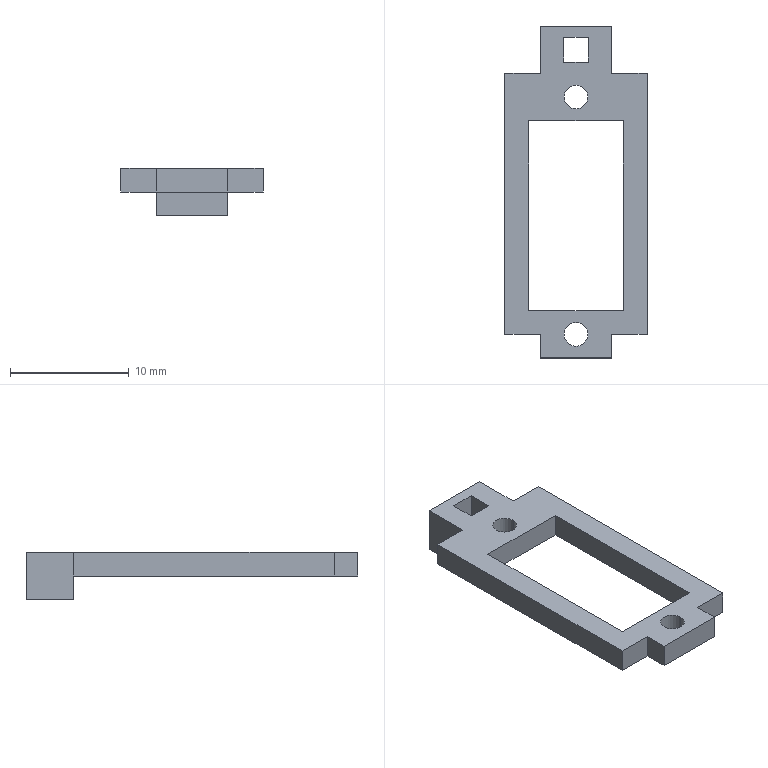Component | SolidWorks | ServoHanger-1 | 1 solid | 28 faces | box 12 x 28 x 4 mm | volume 362 mm3 | plane 24 | cylinder 4 | commonest cylinder face diameters 2 x4
build123d program:
from build123d import *

# Parameters (mm, degrees)
SKETCH1_W           = 6
SKETCH1_H           = 4
SKETCH1_W_2         = 2.1
SKETCH1_H_2         = 2.1
BOSS_EXTRUDE1_DEPTH = 4
SKETCH2_W           = 6
SKETCH2_H           = 24
BOSS_EXTRUDE2_DEPTH = 2
SKETCH3_R           = 1
CUT_EXTRUDE1_DEPTH  = 2
SKETCH5_W           = 3
SKETCH5_H           = 24
BOSS_EXTRUDE3_DEPTH = 2
SKETCH4_W           = 8
SKETCH4_H           = 16
CUT_EXTRUDE2_DEPTH  = 2
SKETCH6_W           = 3
SKETCH6_H           = 2
CUT_EXTRUDE3_DEPTH  = 2


with BuildPart() as part:
    # Sketch1 → Boss-Extrude1 (new body)
    with BuildSketch(Plane.XY):
        Rectangle(SKETCH1_W, SKETCH1_H)
        Rectangle(SKETCH1_W_2, SKETCH1_H_2, mode=Mode.SUBTRACT)
    extrude(amount=BOSS_EXTRUDE1_DEPTH)

    # Sketch2 → Boss-Extrude2 (add)
    with BuildSketch(Plane.XY.offset(4)):
        with Locations((0, -14)):
            Rectangle(SKETCH2_W, SKETCH2_H)
    extrude(amount=-BOSS_EXTRUDE2_DEPTH)

    # Sketch3 → Cut-Extrude1 (cut)
    with BuildSketch(Plane.XY.offset(4)):
        with Locations((0, -4)):
            Circle(SKETCH3_R)
        with Locations(Location((0, -24, 0), (0, 0, 180))):
            Circle(SKETCH3_R)
    extrude(amount=-CUT_EXTRUDE1_DEPTH, mode=Mode.SUBTRACT)

    # Sketch5 → Boss-Extrude3 (add)
    with BuildSketch(Plane(origin=(0, 0, 2), x_dir=(-1, 0, 0), z_dir=(0, 0, -1))):
        with Locations((-4.5, -14)):
            Rectangle(SKETCH5_W, SKETCH5_H)
        with Locations((4.5, -14)):
            Rectangle(SKETCH5_W, SKETCH5_H)
    extrude(amount=-BOSS_EXTRUDE3_DEPTH)

    # Sketch4 → Cut-Extrude2 (cut)
    with BuildSketch(Plane(origin=(0, 0, 2), x_dir=(-1, 0, 0), z_dir=(0, 0, -1))):
        with Locations((0, -14)):
            Rectangle(SKETCH4_W, SKETCH4_H)
    extrude(amount=-CUT_EXTRUDE2_DEPTH, mode=Mode.SUBTRACT)

    # Sketch6 → Cut-Extrude3 (cut)
    with BuildSketch(Plane.XY.offset(4)):
        with Locations((-4.5, -25)):
            Rectangle(SKETCH6_W, SKETCH6_H)
    cut_extrude3 = extrude(amount=-CUT_EXTRUDE3_DEPTH, mode=Mode.SUBTRACT)

    # Mirror1: Cut-Extrude3 across plane
    add(cut_extrude3.mirror(Plane(origin=(0, 0, 0), x_dir=(0, 0, 1), z_dir=(1, 0, 0))), mode=Mode.SUBTRACT)


solid = part.part

# Placed as in the assembly
solid = solid.moved(Location((0.5986, 8.796, -71.03), (0, 0, 0)))
STEP:
#1=COLOUR_RGB('',0.7922,0.8196,0.9333);
#2=FILL_AREA_STYLE_COLOUR('',#1);
#3=FILL_AREA_STYLE('',(#2));
#4=SURFACE_STYLE_FILL_AREA(#3);
#5=SURFACE_SIDE_STYLE('',(#4));
#6=SURFACE_STYLE_USAGE(.BOTH.,#5);
#7=PRESENTATION_STYLE_ASSIGNMENT((#6));
#8=CARTESIAN_POINT('',(-0.0158,0.1888,-2.718));
#9=VERTEX_POINT('',#8);
#10=CARTESIAN_POINT('',(0.06294,0.1888,-2.718));
#11=VERTEX_POINT('',#10);
#12=CARTESIAN_POINT('',(0.02357,0.1888,-2.718));
#13=DIRECTION('',(0.,0.,1.));
#14=DIRECTION('',(1.,0.,0.));
#15=AXIS2_PLACEMENT_3D('',#12,#13,#14);
#16=CIRCLE('',#15,0.03937);
#17=EDGE_CURVE('',#9,#11,#16,.T.);
#18=ORIENTED_EDGE('',*,*,#17,.F.);
#19=CARTESIAN_POINT('',(-0.0158,0.1888,-2.639));
#20=VERTEX_POINT('',#19);
#21=CARTESIAN_POINT('',(-0.0158,0.1888,-2.718));
#22=DIRECTION('',(0.,0.,1.));
#23=VECTOR('',#22,39.37);
#24=LINE('',#21,#23);
#25=EDGE_CURVE('',#9,#20,#24,.T.);
#26=ORIENTED_EDGE('',*,*,#25,.T.);
#27=CARTESIAN_POINT('',(0.06294,0.1888,-2.639));
#28=VERTEX_POINT('',#27);
#29=CARTESIAN_POINT('',(0.02357,0.1888,-2.639));
#30=DIRECTION('',(0.,0.,1.));
#31=DIRECTION('',(1.,0.,0.));
#32=AXIS2_PLACEMENT_3D('',#29,#30,#31);
#33=CIRCLE('',#32,0.03937);
#34=EDGE_CURVE('',#20,#28,#33,.T.);
#35=ORIENTED_EDGE('',*,*,#34,.T.);
#36=CARTESIAN_POINT('',(0.06294,0.1888,-2.718));
#37=DIRECTION('',(0.,0.,1.));
#38=VECTOR('',#37,39.37);
#39=LINE('',#36,#38);
#40=EDGE_CURVE('',#11,#28,#39,.T.);
#41=ORIENTED_EDGE('',*,*,#40,.F.);
#42=EDGE_LOOP('',(#18,#26,#35,#41));
#43=FACE_OUTER_BOUND('',#42,.T.);
#44=CARTESIAN_POINT('',(0.02357,0.1888,-2.718));
#45=DIRECTION('',(0.,0.,1.));
#46=DIRECTION('',(1.,0.,0.));
#47=AXIS2_PLACEMENT_3D('',#44,#45,#46);
#48=CYLINDRICAL_SURFACE('',#47,0.03937);
#49=ADVANCED_FACE('',(#43),#48,.F.);
#50=CARTESIAN_POINT('',(-0.0158,-0.5986,-2.718));
#51=VERTEX_POINT('',#50);
#52=CARTESIAN_POINT('',(0.06294,-0.5986,-2.718));
#53=VERTEX_POINT('',#52);
#54=CARTESIAN_POINT('',(0.02357,-0.5986,-2.718));
#55=DIRECTION('',(0.,0.,1.));
#56=DIRECTION('',(-1.,0.,0.));
#57=AXIS2_PLACEMENT_3D('',#54,#55,#56);
#58=CIRCLE('',#57,0.03937);
#59=EDGE_CURVE('',#51,#53,#58,.T.);
#60=ORIENTED_EDGE('',*,*,#59,.F.);
#61=CARTESIAN_POINT('',(-0.0158,-0.5986,-2.639));
#62=VERTEX_POINT('',#61);
#63=CARTESIAN_POINT('',(-0.0158,-0.5986,-2.718));
#64=DIRECTION('',(0.,0.,1.));
#65=VECTOR('',#64,39.37);
#66=LINE('',#63,#65);
#67=EDGE_CURVE('',#51,#62,#66,.T.);
#68=ORIENTED_EDGE('',*,*,#67,.T.);
#69=CARTESIAN_POINT('',(0.06294,-0.5986,-2.639));
#70=VERTEX_POINT('',#69);
#71=CARTESIAN_POINT('',(0.02357,-0.5986,-2.639));
#72=DIRECTION('',(0.,0.,1.));
#73=DIRECTION('',(-1.,0.,0.));
#74=AXIS2_PLACEMENT_3D('',#71,#72,#73);
#75=CIRCLE('',#74,0.03937);
#76=EDGE_CURVE('',#62,#70,#75,.T.);
#77=ORIENTED_EDGE('',*,*,#76,.T.);
#78=CARTESIAN_POINT('',(0.06294,-0.5986,-2.718));
#79=DIRECTION('',(0.,0.,1.));
#80=VECTOR('',#79,39.37);
#81=LINE('',#78,#80);
#82=EDGE_CURVE('',#53,#70,#81,.T.);
#83=ORIENTED_EDGE('',*,*,#82,.F.);
#84=EDGE_LOOP('',(#60,#68,#77,#83));
#85=FACE_OUTER_BOUND('',#84,.T.);
#86=CARTESIAN_POINT('',(0.02357,-0.5986,-2.718));
#87=DIRECTION('',(0.,0.,1.));
#88=DIRECTION('',(1.,0.,0.));
#89=AXIS2_PLACEMENT_3D('',#86,#87,#88);
#90=CYLINDRICAL_SURFACE('',#89,0.03937);
#91=ADVANCED_FACE('',(#85),#90,.F.);
#92=CARTESIAN_POINT('',(0.06491,0.305,-2.639));
#93=VERTEX_POINT('',#92);
#94=CARTESIAN_POINT('',(0.06491,0.3876,-2.639));
#95=VERTEX_POINT('',#94);
#96=CARTESIAN_POINT('',(0.06491,0.305,-2.639));
#97=DIRECTION('',(0.,1.,0.));
#98=VECTOR('',#97,39.37);
#99=LINE('',#96,#98);
#100=EDGE_CURVE('',#93,#95,#99,.T.);
#101=ORIENTED_EDGE('',*,*,#100,.F.);
#102=CARTESIAN_POINT('',(-0.01777,0.305,-2.639));
#103=VERTEX_POINT('',#102);
#104=CARTESIAN_POINT('',(-0.01777,0.305,-2.639));
#105=DIRECTION('',(1.,0.,0.));
#106=VECTOR('',#105,39.37);
#107=LINE('',#104,#106);
#108=EDGE_CURVE('',#103,#93,#107,.T.);
#109=ORIENTED_EDGE('',*,*,#108,.F.);
#110=CARTESIAN_POINT('',(-0.01777,0.3876,-2.639));
#111=VERTEX_POINT('',#110);
#112=CARTESIAN_POINT('',(-0.01777,0.305,-2.639));
#113=DIRECTION('',(0.,-1.,0.));
#114=VECTOR('',#113,39.37);
#115=LINE('',#112,#114);
#116=EDGE_CURVE('',#111,#103,#115,.T.);
#117=ORIENTED_EDGE('',*,*,#116,.F.);
#118=CARTESIAN_POINT('',(-0.01777,0.3876,-2.639));
#119=DIRECTION('',(-1.,0.,0.));
#120=VECTOR('',#119,39.37);
#121=LINE('',#118,#120);
#122=EDGE_CURVE('',#95,#111,#121,.T.);
#123=ORIENTED_EDGE('',*,*,#122,.F.);
#124=EDGE_LOOP('',(#101,#109,#117,#123));
#125=FACE_BOUND('',#124,.T.);
#126=CARTESIAN_POINT('',(0.02357,-0.5986,-2.639));
#127=DIRECTION('',(0.,0.,1.));
#128=DIRECTION('',(-1.,0.,0.));
#129=AXIS2_PLACEMENT_3D('',#126,#127,#128);
#130=CIRCLE('',#129,0.03937);
#131=EDGE_CURVE('',#70,#62,#130,.T.);
#132=ORIENTED_EDGE('',*,*,#131,.F.);
#133=ORIENTED_EDGE('',*,*,#76,.F.);
#134=EDGE_LOOP('',(#132,#133));
#135=FACE_BOUND('',#134,.T.);
#136=CARTESIAN_POINT('',(0.02357,0.1888,-2.639));
#137=DIRECTION('',(0.,0.,1.));
#138=DIRECTION('',(1.,0.,0.));
#139=AXIS2_PLACEMENT_3D('',#136,#137,#138);
#140=CIRCLE('',#139,0.03937);
#141=EDGE_CURVE('',#28,#20,#140,.T.);
#142=ORIENTED_EDGE('',*,*,#141,.F.);
#143=ORIENTED_EDGE('',*,*,#34,.F.);
#144=EDGE_LOOP('',(#142,#143));
#145=FACE_BOUND('',#144,.T.);
#146=CARTESIAN_POINT('',(-0.1339,0.1101,-2.639));
#147=VERTEX_POINT('',#146);
#148=CARTESIAN_POINT('',(0.181,0.1101,-2.639));
#149=VERTEX_POINT('',#148);
#150=CARTESIAN_POINT('',(0.181,0.1101,-2.639));
#151=DIRECTION('',(1.,0.,0.));
#152=VECTOR('',#151,39.37);
#153=LINE('',#150,#152);
#154=EDGE_CURVE('',#147,#149,#153,.T.);
#155=ORIENTED_EDGE('',*,*,#154,.T.);
#156=CARTESIAN_POINT('',(0.181,-0.5198,-2.639));
#157=VERTEX_POINT('',#156);
#158=CARTESIAN_POINT('',(0.181,-0.5198,-2.639));
#159=DIRECTION('',(0.,-1.,0.));
#160=VECTOR('',#159,39.37);
#161=LINE('',#158,#160);
#162=EDGE_CURVE('',#149,#157,#161,.T.);
#163=ORIENTED_EDGE('',*,*,#162,.T.);
#164=CARTESIAN_POINT('',(-0.1339,-0.5198,-2.639));
#165=VERTEX_POINT('',#164);
#166=CARTESIAN_POINT('',(0.181,-0.5198,-2.639));
#167=DIRECTION('',(-1.,0.,0.));
#168=VECTOR('',#167,39.37);
#169=LINE('',#166,#168);
#170=EDGE_CURVE('',#157,#165,#169,.T.);
#171=ORIENTED_EDGE('',*,*,#170,.T.);
#172=CARTESIAN_POINT('',(-0.1339,-0.5198,-2.639));
#173=DIRECTION('',(0.,1.,0.));
#174=VECTOR('',#173,39.37);
#175=LINE('',#172,#174);
#176=EDGE_CURVE('',#165,#147,#175,.T.);
#177=ORIENTED_EDGE('',*,*,#176,.T.);
#178=EDGE_LOOP('',(#155,#163,#171,#177));
#179=FACE_BOUND('',#178,.T.);
#180=CARTESIAN_POINT('',(0.1417,-0.6773,-2.639));
#181=VERTEX_POINT('',#180);
#182=CARTESIAN_POINT('',(0.1417,-0.5986,-2.639));
#183=VERTEX_POINT('',#182);
#184=CARTESIAN_POINT('',(0.1417,-0.6773,-2.639));
#185=DIRECTION('',(0.,1.,0.));
#186=VECTOR('',#185,39.37);
#187=LINE('',#184,#186);
#188=EDGE_CURVE('',#181,#183,#187,.T.);
#189=ORIENTED_EDGE('',*,*,#188,.T.);
#190=CARTESIAN_POINT('',(0.2598,-0.5986,-2.639));
#191=VERTEX_POINT('',#190);
#192=CARTESIAN_POINT('',(0.2598,-0.5986,-2.639));
#193=DIRECTION('',(1.,0.,0.));
#194=VECTOR('',#193,39.37);
#195=LINE('',#192,#194);
#196=EDGE_CURVE('',#183,#191,#195,.T.);
#197=ORIENTED_EDGE('',*,*,#196,.T.);
#198=CARTESIAN_POINT('',(0.2598,0.2676,-2.639));
#199=VERTEX_POINT('',#198);
#200=CARTESIAN_POINT('',(0.2598,0.2676,-2.639));
#201=DIRECTION('',(0.,1.,0.));
#202=VECTOR('',#201,39.37);
#203=LINE('',#200,#202);
#204=EDGE_CURVE('',#191,#199,#203,.T.);
#205=ORIENTED_EDGE('',*,*,#204,.T.);
#206=CARTESIAN_POINT('',(0.1417,0.2676,-2.639));
#207=VERTEX_POINT('',#206);
#208=CARTESIAN_POINT('',(0.1417,0.2676,-2.639));
#209=DIRECTION('',(-1.,0.,0.));
#210=VECTOR('',#209,39.37);
#211=LINE('',#208,#210);
#212=EDGE_CURVE('',#199,#207,#211,.T.);
#213=ORIENTED_EDGE('',*,*,#212,.T.);
#214=CARTESIAN_POINT('',(0.1417,0.425,-2.639));
#215=VERTEX_POINT('',#214);
#216=CARTESIAN_POINT('',(0.1417,0.2676,-2.639));
#217=DIRECTION('',(0.,1.,0.));
#218=VECTOR('',#217,39.37);
#219=LINE('',#216,#218);
#220=EDGE_CURVE('',#207,#215,#219,.T.);
#221=ORIENTED_EDGE('',*,*,#220,.T.);
#222=CARTESIAN_POINT('',(-0.09454,0.425,-2.639));
#223=VERTEX_POINT('',#222);
#224=CARTESIAN_POINT('',(-0.09454,0.425,-2.639));
#225=DIRECTION('',(-1.,0.,0.));
#226=VECTOR('',#225,39.37);
#227=LINE('',#224,#226);
#228=EDGE_CURVE('',#215,#223,#227,.T.);
#229=ORIENTED_EDGE('',*,*,#228,.T.);
#230=CARTESIAN_POINT('',(-0.09454,0.2676,-2.639));
#231=VERTEX_POINT('',#230);
#232=CARTESIAN_POINT('',(-0.09454,0.2676,-2.639));
#233=DIRECTION('',(0.,-1.,0.));
#234=VECTOR('',#233,39.37);
#235=LINE('',#232,#234);
#236=EDGE_CURVE('',#223,#231,#235,.T.);
#237=ORIENTED_EDGE('',*,*,#236,.T.);
#238=CARTESIAN_POINT('',(-0.2127,0.2676,-2.639));
#239=VERTEX_POINT('',#238);
#240=CARTESIAN_POINT('',(-0.09454,0.2676,-2.639));
#241=DIRECTION('',(-1.,0.,0.));
#242=VECTOR('',#241,39.37);
#243=LINE('',#240,#242);
#244=EDGE_CURVE('',#231,#239,#243,.T.);
#245=ORIENTED_EDGE('',*,*,#244,.T.);
#246=CARTESIAN_POINT('',(-0.2127,-0.5986,-2.639));
#247=VERTEX_POINT('',#246);
#248=CARTESIAN_POINT('',(-0.2127,0.2676,-2.639));
#249=DIRECTION('',(-0.,-1.,0.));
#250=VECTOR('',#249,39.37);
#251=LINE('',#248,#250);
#252=EDGE_CURVE('',#239,#247,#251,.T.);
#253=ORIENTED_EDGE('',*,*,#252,.T.);
#254=CARTESIAN_POINT('',(-0.09454,-0.5986,-2.639));
#255=VERTEX_POINT('',#254);
#256=CARTESIAN_POINT('',(-0.2127,-0.5986,-2.639));
#257=DIRECTION('',(-1.,0.,0.));
#258=VECTOR('',#257,39.37);
#259=LINE('',#256,#258);
#260=EDGE_CURVE('',#255,#247,#259,.T.);
#261=ORIENTED_EDGE('',*,*,#260,.F.);
#262=CARTESIAN_POINT('',(-0.09454,-0.6773,-2.639));
#263=VERTEX_POINT('',#262);
#264=CARTESIAN_POINT('',(-0.09454,-0.6773,-2.639));
#265=DIRECTION('',(0.,1.,0.));
#266=VECTOR('',#265,39.37);
#267=LINE('',#264,#266);
#268=EDGE_CURVE('',#263,#255,#267,.T.);
#269=ORIENTED_EDGE('',*,*,#268,.F.);
#270=CARTESIAN_POINT('',(-0.09454,-0.6773,-2.639));
#271=DIRECTION('',(1.,0.,0.));
#272=VECTOR('',#271,39.37);
#273=LINE('',#270,#272);
#274=EDGE_CURVE('',#263,#181,#273,.T.);
#275=ORIENTED_EDGE('',*,*,#274,.T.);
#276=EDGE_LOOP('',(#189,#197,#205,#213,#221,#229,#237,#245,#253,#261,#269,#275));
#277=FACE_OUTER_BOUND('',#276,.T.);
#278=CARTESIAN_POINT('',(0.02357,0.3463,-2.639));
#279=DIRECTION('',(0.,0.,-1.));
#280=DIRECTION('',(-1.,0.,0.));
#281=AXIS2_PLACEMENT_3D('',#278,#279,#280);
#282=PLANE('',#281);
#283=ADVANCED_FACE('',(#125,#135,#145,#179,#277),#282,.F.);
#284=CARTESIAN_POINT('',(-0.09454,-0.6773,-2.718));
#285=VERTEX_POINT('',#284);
#286=CARTESIAN_POINT('',(0.1417,-0.6773,-2.718));
#287=VERTEX_POINT('',#286);
#288=CARTESIAN_POINT('',(-0.09454,-0.6773,-2.718));
#289=DIRECTION('',(1.,0.,0.));
#290=VECTOR('',#289,39.37);
#291=LINE('',#288,#290);
#292=EDGE_CURVE('',#285,#287,#291,.T.);
#293=ORIENTED_EDGE('',*,*,#292,.T.);
#294=CARTESIAN_POINT('',(0.1417,-0.6773,-2.718));
#295=DIRECTION('',(0.,0.,1.));
#296=VECTOR('',#295,39.37);
#297=LINE('',#294,#296);
#298=EDGE_CURVE('',#287,#181,#297,.T.);
#299=ORIENTED_EDGE('',*,*,#298,.T.);
#300=ORIENTED_EDGE('',*,*,#274,.F.);
#301=CARTESIAN_POINT('',(-0.09454,-0.6773,-2.718));
#302=DIRECTION('',(0.,0.,1.));
#303=VECTOR('',#302,39.37);
#304=LINE('',#301,#303);
#305=EDGE_CURVE('',#285,#263,#304,.T.);
#306=ORIENTED_EDGE('',*,*,#305,.F.);
#307=EDGE_LOOP('',(#293,#299,#300,#306));
#308=FACE_OUTER_BOUND('',#307,.T.);
#309=CARTESIAN_POINT('',(-0.09454,-0.6773,-2.718));
#310=DIRECTION('',(0.,-1.,0.));
#311=DIRECTION('',(0.,0.,-1.));
#312=AXIS2_PLACEMENT_3D('',#309,#310,#311);
#313=PLANE('',#312);
#314=ADVANCED_FACE('',(#308),#313,.T.);
#315=CARTESIAN_POINT('',(0.02357,-0.5986,-2.718));
#316=DIRECTION('',(0.,0.,1.));
#317=DIRECTION('',(-1.,0.,0.));
#318=AXIS2_PLACEMENT_3D('',#315,#316,#317);
#319=CIRCLE('',#318,0.03937);
#320=EDGE_CURVE('',#53,#51,#319,.T.);
#321=ORIENTED_EDGE('',*,*,#320,.T.);
#322=ORIENTED_EDGE('',*,*,#59,.T.);
#323=EDGE_LOOP('',(#321,#322));
#324=FACE_BOUND('',#323,.T.);
#325=CARTESIAN_POINT('',(0.02357,0.1888,-2.718));
#326=DIRECTION('',(0.,0.,1.));
#327=DIRECTION('',(1.,0.,0.));
#328=AXIS2_PLACEMENT_3D('',#325,#326,#327);
#329=CIRCLE('',#328,0.03937);
#330=EDGE_CURVE('',#11,#9,#329,.T.);
#331=ORIENTED_EDGE('',*,*,#330,.T.);
#332=ORIENTED_EDGE('',*,*,#17,.T.);
#333=EDGE_LOOP('',(#331,#332));
#334=FACE_BOUND('',#333,.T.);
#335=CARTESIAN_POINT('',(0.181,-0.5198,-2.718));
#336=VERTEX_POINT('',#335);
#337=CARTESIAN_POINT('',(-0.1339,-0.5198,-2.718));
#338=VERTEX_POINT('',#337);
#339=CARTESIAN_POINT('',(0.181,-0.5198,-2.718));
#340=DIRECTION('',(-1.,0.,0.));
#341=VECTOR('',#340,39.37);
#342=LINE('',#339,#341);
#343=EDGE_CURVE('',#336,#338,#342,.T.);
#344=ORIENTED_EDGE('',*,*,#343,.F.);
#345=CARTESIAN_POINT('',(0.181,0.1101,-2.718));
#346=VERTEX_POINT('',#345);
#347=CARTESIAN_POINT('',(0.181,-0.5198,-2.718));
#348=DIRECTION('',(0.,-1.,0.));
#349=VECTOR('',#348,39.37);
#350=LINE('',#347,#349);
#351=EDGE_CURVE('',#346,#336,#350,.T.);
#352=ORIENTED_EDGE('',*,*,#351,.F.);
#353=CARTESIAN_POINT('',(-0.1339,0.1101,-2.718));
#354=VERTEX_POINT('',#353);
#355=CARTESIAN_POINT('',(0.181,0.1101,-2.718));
#356=DIRECTION('',(1.,0.,0.));
#357=VECTOR('',#356,39.37);
#358=LINE('',#355,#357);
#359=EDGE_CURVE('',#354,#346,#358,.T.);
#360=ORIENTED_EDGE('',*,*,#359,.F.);
#361=CARTESIAN_POINT('',(-0.1339,-0.5198,-2.718));
#362=DIRECTION('',(0.,1.,0.));
#363=VECTOR('',#362,39.37);
#364=LINE('',#361,#363);
#365=EDGE_CURVE('',#338,#354,#364,.T.);
#366=ORIENTED_EDGE('',*,*,#365,.F.);
#367=EDGE_LOOP('',(#344,#352,#360,#366));
#368=FACE_BOUND('',#367,.T.);
#369=CARTESIAN_POINT('',(0.1417,-0.5986,-2.718));
#370=VERTEX_POINT('',#369);
#371=CARTESIAN_POINT('',(0.1417,-0.6773,-2.718));
#372=DIRECTION('',(0.,1.,0.));
#373=VECTOR('',#372,39.37);
#374=LINE('',#371,#373);
#375=EDGE_CURVE('',#287,#370,#374,.T.);
#376=ORIENTED_EDGE('',*,*,#375,.F.);
#377=ORIENTED_EDGE('',*,*,#292,.F.);
#378=CARTESIAN_POINT('',(-0.09454,-0.5986,-2.718));
#379=VERTEX_POINT('',#378);
#380=CARTESIAN_POINT('',(-0.09454,-0.6773,-2.718));
#381=DIRECTION('',(0.,1.,0.));
#382=VECTOR('',#381,39.37);
#383=LINE('',#380,#382);
#384=EDGE_CURVE('',#285,#379,#383,.T.);
#385=ORIENTED_EDGE('',*,*,#384,.T.);
#386=CARTESIAN_POINT('',(-0.2127,-0.5986,-2.718));
#387=VERTEX_POINT('',#386);
#388=CARTESIAN_POINT('',(-0.2127,-0.5986,-2.718));
#389=DIRECTION('',(-1.,0.,0.));
#390=VECTOR('',#389,39.37);
#391=LINE('',#388,#390);
#392=EDGE_CURVE('',#379,#387,#391,.T.);
#393=ORIENTED_EDGE('',*,*,#392,.T.);
#394=CARTESIAN_POINT('',(-0.2127,0.2676,-2.718));
#395=VERTEX_POINT('',#394);
#396=CARTESIAN_POINT('',(-0.2127,0.2676,-2.718));
#397=DIRECTION('',(0.,1.,0.));
#398=VECTOR('',#397,39.37);
#399=LINE('',#396,#398);
#400=EDGE_CURVE('',#387,#395,#399,.T.);
#401=ORIENTED_EDGE('',*,*,#400,.T.);
#402=CARTESIAN_POINT('',(-0.09454,0.2676,-2.718));
#403=VERTEX_POINT('',#402);
#404=CARTESIAN_POINT('',(-0.09454,0.2676,-2.718));
#405=DIRECTION('',(1.,-0.,0.));
#406=VECTOR('',#405,39.37);
#407=LINE('',#404,#406);
#408=EDGE_CURVE('',#395,#403,#407,.T.);
#409=ORIENTED_EDGE('',*,*,#408,.T.);
#410=CARTESIAN_POINT('',(0.1417,0.2676,-2.718));
#411=VERTEX_POINT('',#410);
#412=CARTESIAN_POINT('',(-0.09454,0.2676,-2.718));
#413=DIRECTION('',(-1.,0.,0.));
#414=VECTOR('',#413,39.37);
#415=LINE('',#412,#414);
#416=EDGE_CURVE('',#411,#403,#415,.T.);
#417=ORIENTED_EDGE('',*,*,#416,.F.);
#418=CARTESIAN_POINT('',(0.2598,0.2676,-2.718));
#419=VERTEX_POINT('',#418);
#420=CARTESIAN_POINT('',(0.1417,0.2676,-2.718));
#421=DIRECTION('',(1.,0.,0.));
#422=VECTOR('',#421,39.37);
#423=LINE('',#420,#422);
#424=EDGE_CURVE('',#411,#419,#423,.T.);
#425=ORIENTED_EDGE('',*,*,#424,.T.);
#426=CARTESIAN_POINT('',(0.2598,-0.5986,-2.718));
#427=VERTEX_POINT('',#426);
#428=CARTESIAN_POINT('',(0.2598,0.2676,-2.718));
#429=DIRECTION('',(-0.,-1.,0.));
#430=VECTOR('',#429,39.37);
#431=LINE('',#428,#430);
#432=EDGE_CURVE('',#419,#427,#431,.T.);
#433=ORIENTED_EDGE('',*,*,#432,.T.);
#434=CARTESIAN_POINT('',(0.2598,-0.5986,-2.718));
#435=DIRECTION('',(1.,0.,0.));
#436=VECTOR('',#435,39.37);
#437=LINE('',#434,#436);
#438=EDGE_CURVE('',#370,#427,#437,.T.);
#439=ORIENTED_EDGE('',*,*,#438,.F.);
#440=EDGE_LOOP('',(#376,#377,#385,#393,#401,#409,#417,#425,#433,#439));
#441=FACE_OUTER_BOUND('',#440,.T.);
#442=CARTESIAN_POINT('',(0.02357,0.3463,-2.718));
#443=DIRECTION('',(0.,0.,1.));
#444=DIRECTION('',(1.,0.,0.));
#445=AXIS2_PLACEMENT_3D('',#442,#443,#444);
#446=PLANE('',#445);
#447=ADVANCED_FACE('',(#324,#334,#368,#441),#446,.F.);
#448=ORIENTED_EDGE('',*,*,#204,.F.);
#449=CARTESIAN_POINT('',(0.2598,-0.5986,-2.718));
#450=DIRECTION('',(0.,0.,1.));
#451=VECTOR('',#450,39.37);
#452=LINE('',#449,#451);
#453=EDGE_CURVE('',#427,#191,#452,.T.);
#454=ORIENTED_EDGE('',*,*,#453,.F.);
#455=ORIENTED_EDGE('',*,*,#432,.F.);
#456=CARTESIAN_POINT('',(0.2598,0.2676,-1.687));
#457=DIRECTION('',(0.,0.,-1.));
#458=VECTOR('',#457,39.37);
#459=LINE('',#456,#458);
#460=EDGE_CURVE('',#199,#419,#459,.T.);
#461=ORIENTED_EDGE('',*,*,#460,.F.);
#462=EDGE_LOOP('',(#448,#454,#455,#461));
#463=FACE_OUTER_BOUND('',#462,.T.);
#464=CARTESIAN_POINT('',(0.2598,0.2676,-1.687));
#465=DIRECTION('',(1.,-0.,0.));
#466=DIRECTION('',(0.,1.,0.));
#467=AXIS2_PLACEMENT_3D('',#464,#465,#466);
#468=PLANE('',#467);
#469=ADVANCED_FACE('',(#463),#468,.T.);
#470=CARTESIAN_POINT('',(-0.09454,0.2676,-1.687));
#471=DIRECTION('',(0.,0.,-1.));
#472=VECTOR('',#471,39.37);
#473=LINE('',#470,#472);
#474=EDGE_CURVE('',#231,#403,#473,.T.);
#475=ORIENTED_EDGE('',*,*,#474,.F.);
#476=ORIENTED_EDGE('',*,*,#236,.F.);
#477=CARTESIAN_POINT('',(-0.09454,0.425,-2.796));
#478=VERTEX_POINT('',#477);
#479=CARTESIAN_POINT('',(-0.09454,0.425,-2.639));
#480=DIRECTION('',(0.,0.,-1.));
#481=VECTOR('',#480,39.37);
#482=LINE('',#479,#481);
#483=EDGE_CURVE('',#223,#478,#482,.T.);
#484=ORIENTED_EDGE('',*,*,#483,.T.);
#485=CARTESIAN_POINT('',(-0.09454,0.2676,-2.796));
#486=VERTEX_POINT('',#485);
#487=CARTESIAN_POINT('',(-0.09454,0.2676,-2.796));
#488=DIRECTION('',(0.,-1.,0.));
#489=VECTOR('',#488,39.37);
#490=LINE('',#487,#489);
#491=EDGE_CURVE('',#478,#486,#490,.T.);
#492=ORIENTED_EDGE('',*,*,#491,.T.);
#493=CARTESIAN_POINT('',(-0.09454,0.2676,-2.639));
#494=DIRECTION('',(0.,0.,-1.));
#495=VECTOR('',#494,39.37);
#496=LINE('',#493,#495);
#497=EDGE_CURVE('',#403,#486,#496,.T.);
#498=ORIENTED_EDGE('',*,*,#497,.F.);
#499=EDGE_LOOP('',(#475,#476,#484,#492,#498));
#500=FACE_OUTER_BOUND('',#499,.T.);
#501=CARTESIAN_POINT('',(-0.09454,0.2676,-2.639));
#502=DIRECTION('',(1.,0.,0.));
#503=DIRECTION('',(0.,0.,-1.));
#504=AXIS2_PLACEMENT_3D('',#501,#502,#503);
#505=PLANE('',#504);
#506=ADVANCED_FACE('',(#500),#505,.F.);
#507=CARTESIAN_POINT('',(0.1417,0.2676,-2.796));
#508=VERTEX_POINT('',#507);
#509=CARTESIAN_POINT('',(0.1417,0.425,-2.796));
#510=VERTEX_POINT('',#509);
#511=CARTESIAN_POINT('',(0.1417,0.2676,-2.796));
#512=DIRECTION('',(0.,1.,0.));
#513=VECTOR('',#512,39.37);
#514=LINE('',#511,#513);
#515=EDGE_CURVE('',#508,#510,#514,.T.);
#516=ORIENTED_EDGE('',*,*,#515,.F.);
#517=CARTESIAN_POINT('',(-0.09454,0.2676,-2.796));
#518=DIRECTION('',(1.,0.,0.));
#519=VECTOR('',#518,39.37);
#520=LINE('',#517,#519);
#521=EDGE_CURVE('',#486,#508,#520,.T.);
#522=ORIENTED_EDGE('',*,*,#521,.F.);
#523=ORIENTED_EDGE('',*,*,#491,.F.);
#524=CARTESIAN_POINT('',(-0.09454,0.425,-2.796));
#525=DIRECTION('',(-1.,0.,0.));
#526=VECTOR('',#525,39.37);
#527=LINE('',#524,#526);
#528=EDGE_CURVE('',#510,#478,#527,.T.);
#529=ORIENTED_EDGE('',*,*,#528,.F.);
#530=EDGE_LOOP('',(#516,#522,#523,#529));
#531=FACE_OUTER_BOUND('',#530,.T.);
#532=CARTESIAN_POINT('',(-0.01777,0.305,-2.796));
#533=VERTEX_POINT('',#532);
#534=CARTESIAN_POINT('',(0.06491,0.305,-2.796));
#535=VERTEX_POINT('',#534);
#536=CARTESIAN_POINT('',(-0.01777,0.305,-2.796));
#537=DIRECTION('',(1.,0.,0.));
#538=VECTOR('',#537,39.37);
#539=LINE('',#536,#538);
#540=EDGE_CURVE('',#533,#535,#539,.T.);
#541=ORIENTED_EDGE('',*,*,#540,.T.);
#542=CARTESIAN_POINT('',(0.06491,0.3876,-2.796));
#543=VERTEX_POINT('',#542);
#544=CARTESIAN_POINT('',(0.06491,0.305,-2.796));
#545=DIRECTION('',(0.,1.,0.));
#546=VECTOR('',#545,39.37);
#547=LINE('',#544,#546);
#548=EDGE_CURVE('',#535,#543,#547,.T.);
#549=ORIENTED_EDGE('',*,*,#548,.T.);
#550=CARTESIAN_POINT('',(-0.01777,0.3876,-2.796));
#551=VERTEX_POINT('',#550);
#552=CARTESIAN_POINT('',(-0.01777,0.3876,-2.796));
#553=DIRECTION('',(-1.,0.,0.));
#554=VECTOR('',#553,39.37);
#555=LINE('',#552,#554);
#556=EDGE_CURVE('',#543,#551,#555,.T.);
#557=ORIENTED_EDGE('',*,*,#556,.T.);
#558=CARTESIAN_POINT('',(-0.01777,0.305,-2.796));
#559=DIRECTION('',(0.,-1.,0.));
#560=VECTOR('',#559,39.37);
#561=LINE('',#558,#560);
#562=EDGE_CURVE('',#551,#533,#561,.T.);
#563=ORIENTED_EDGE('',*,*,#562,.T.);
#564=EDGE_LOOP('',(#541,#549,#557,#563));
#565=FACE_BOUND('',#564,.T.);
#566=CARTESIAN_POINT('',(0.02357,0.3463,-2.796));
#567=DIRECTION('',(0.,0.,-1.));
#568=DIRECTION('',(-1.,0.,0.));
#569=AXIS2_PLACEMENT_3D('',#566,#567,#568);
#570=PLANE('',#569);
#571=ADVANCED_FACE('',(#531,#565),#570,.T.);
#572=ORIENTED_EDGE('',*,*,#220,.F.);
#573=CARTESIAN_POINT('',(0.1417,0.2676,-1.687));
#574=DIRECTION('',(0.,0.,-1.));
#575=VECTOR('',#574,39.37);
#576=LINE('',#573,#575);
#577=EDGE_CURVE('',#207,#411,#576,.T.);
#578=ORIENTED_EDGE('',*,*,#577,.T.);
#579=CARTESIAN_POINT('',(0.1417,0.2676,-2.639));
#580=DIRECTION('',(0.,0.,-1.));
#581=VECTOR('',#580,39.37);
#582=LINE('',#579,#581);
#583=EDGE_CURVE('',#411,#508,#582,.T.);
#584=ORIENTED_EDGE('',*,*,#583,.T.);
#585=ORIENTED_EDGE('',*,*,#515,.T.);
#586=CARTESIAN_POINT('',(0.1417,0.425,-2.639));
#587=DIRECTION('',(0.,0.,-1.));
#588=VECTOR('',#587,39.37);
#589=LINE('',#586,#588);
#590=EDGE_CURVE('',#215,#510,#589,.T.);
#591=ORIENTED_EDGE('',*,*,#590,.F.);
#592=EDGE_LOOP('',(#572,#578,#584,#585,#591));
#593=FACE_OUTER_BOUND('',#592,.T.);
#594=CARTESIAN_POINT('',(0.1417,0.2676,-2.639));
#595=DIRECTION('',(-1.,0.,0.));
#596=DIRECTION('',(0.,0.,1.));
#597=AXIS2_PLACEMENT_3D('',#594,#595,#596);
#598=PLANE('',#597);
#599=ADVANCED_FACE('',(#593),#598,.F.);
#600=ORIENTED_EDGE('',*,*,#528,.T.);
#601=ORIENTED_EDGE('',*,*,#483,.F.);
#602=ORIENTED_EDGE('',*,*,#228,.F.);
#603=ORIENTED_EDGE('',*,*,#590,.T.);
#604=EDGE_LOOP('',(#600,#601,#602,#603));
#605=FACE_OUTER_BOUND('',#604,.T.);
#606=CARTESIAN_POINT('',(-0.09454,0.425,-2.639));
#607=DIRECTION('',(0.,-1.,0.));
#608=DIRECTION('',(0.,0.,-1.));
#609=AXIS2_PLACEMENT_3D('',#606,#607,#608);
#610=PLANE('',#609);
#611=ADVANCED_FACE('',(#605),#610,.F.);
#612=ORIENTED_EDGE('',*,*,#583,.F.);
#613=ORIENTED_EDGE('',*,*,#416,.T.);
#614=ORIENTED_EDGE('',*,*,#497,.T.);
#615=ORIENTED_EDGE('',*,*,#521,.T.);
#616=EDGE_LOOP('',(#612,#613,#614,#615));
#617=FACE_OUTER_BOUND('',#616,.T.);
#618=CARTESIAN_POINT('',(-0.09454,0.2676,-2.639));
#619=DIRECTION('',(0.,1.,0.));
#620=DIRECTION('',(0.,0.,1.));
#621=AXIS2_PLACEMENT_3D('',#618,#619,#620);
#622=PLANE('',#621);
#623=ADVANCED_FACE('',(#617),#622,.F.);
#624=ORIENTED_EDGE('',*,*,#548,.F.);
#625=CARTESIAN_POINT('',(0.06491,0.305,-2.639));
#626=DIRECTION('',(0.,0.,-1.));
#627=VECTOR('',#626,39.37);
#628=LINE('',#625,#627);
#629=EDGE_CURVE('',#93,#535,#628,.T.);
#630=ORIENTED_EDGE('',*,*,#629,.F.);
#631=ORIENTED_EDGE('',*,*,#100,.T.);
#632=CARTESIAN_POINT('',(0.06491,0.3876,-2.639));
#633=DIRECTION('',(0.,0.,-1.));
#634=VECTOR('',#633,39.37);
#635=LINE('',#632,#634);
#636=EDGE_CURVE('',#95,#543,#635,.T.);
#637=ORIENTED_EDGE('',*,*,#636,.T.);
#638=EDGE_LOOP('',(#624,#630,#631,#637));
#639=FACE_OUTER_BOUND('',#638,.T.);
#640=CARTESIAN_POINT('',(0.06491,0.305,-2.639));
#641=DIRECTION('',(-1.,0.,0.));
#642=DIRECTION('',(0.,0.,1.));
#643=AXIS2_PLACEMENT_3D('',#640,#641,#642);
#644=PLANE('',#643);
#645=ADVANCED_FACE('',(#639),#644,.T.);
#646=ORIENTED_EDGE('',*,*,#556,.F.);
#647=ORIENTED_EDGE('',*,*,#636,.F.);
#648=ORIENTED_EDGE('',*,*,#122,.T.);
#649=CARTESIAN_POINT('',(-0.01777,0.3876,-2.639));
#650=DIRECTION('',(0.,0.,-1.));
#651=VECTOR('',#650,39.37);
#652=LINE('',#649,#651);
#653=EDGE_CURVE('',#111,#551,#652,.T.);
#654=ORIENTED_EDGE('',*,*,#653,.T.);
#655=EDGE_LOOP('',(#646,#647,#648,#654));
#656=FACE_OUTER_BOUND('',#655,.T.);
#657=CARTESIAN_POINT('',(-0.01777,0.3876,-2.639));
#658=DIRECTION('',(0.,-1.,0.));
#659=DIRECTION('',(0.,0.,-1.));
#660=AXIS2_PLACEMENT_3D('',#657,#658,#659);
#661=PLANE('',#660);
#662=ADVANCED_FACE('',(#656),#661,.T.);
#663=ORIENTED_EDGE('',*,*,#562,.F.);
#664=ORIENTED_EDGE('',*,*,#653,.F.);
#665=ORIENTED_EDGE('',*,*,#116,.T.);
#666=CARTESIAN_POINT('',(-0.01777,0.305,-2.639));
#667=DIRECTION('',(0.,0.,-1.));
#668=VECTOR('',#667,39.37);
#669=LINE('',#666,#668);
#670=EDGE_CURVE('',#103,#533,#669,.T.);
#671=ORIENTED_EDGE('',*,*,#670,.T.);
#672=EDGE_LOOP('',(#663,#664,#665,#671));
#673=FACE_OUTER_BOUND('',#672,.T.);
#674=CARTESIAN_POINT('',(-0.01777,0.305,-2.639));
#675=DIRECTION('',(1.,0.,0.));
#676=DIRECTION('',(0.,0.,-1.));
#677=AXIS2_PLACEMENT_3D('',#674,#675,#676);
#678=PLANE('',#677);
#679=ADVANCED_FACE('',(#673),#678,.T.);
#680=ORIENTED_EDGE('',*,*,#540,.F.);
#681=ORIENTED_EDGE('',*,*,#670,.F.);
#682=ORIENTED_EDGE('',*,*,#108,.T.);
#683=ORIENTED_EDGE('',*,*,#629,.T.);
#684=EDGE_LOOP('',(#680,#681,#682,#683));
#685=FACE_OUTER_BOUND('',#684,.T.);
#686=CARTESIAN_POINT('',(-0.01777,0.305,-2.639));
#687=DIRECTION('',(0.,1.,0.));
#688=DIRECTION('',(0.,0.,1.));
#689=AXIS2_PLACEMENT_3D('',#686,#687,#688);
#690=PLANE('',#689);
#691=ADVANCED_FACE('',(#685),#690,.T.);
#692=ORIENTED_EDGE('',*,*,#67,.F.);
#693=ORIENTED_EDGE('',*,*,#320,.F.);
#694=ORIENTED_EDGE('',*,*,#82,.T.);
#695=ORIENTED_EDGE('',*,*,#131,.T.);
#696=EDGE_LOOP('',(#692,#693,#694,#695));
#697=FACE_OUTER_BOUND('',#696,.T.);
#698=CARTESIAN_POINT('',(0.02357,-0.5986,-2.718));
#699=DIRECTION('',(0.,0.,1.));
#700=DIRECTION('',(1.,0.,0.));
#701=AXIS2_PLACEMENT_3D('',#698,#699,#700);
#702=CYLINDRICAL_SURFACE('',#701,0.03937);
#703=ADVANCED_FACE('',(#697),#702,.F.);
#704=ORIENTED_EDGE('',*,*,#25,.F.);
#705=ORIENTED_EDGE('',*,*,#330,.F.);
#706=ORIENTED_EDGE('',*,*,#40,.T.);
#707=ORIENTED_EDGE('',*,*,#141,.T.);
#708=EDGE_LOOP('',(#704,#705,#706,#707));
#709=FACE_OUTER_BOUND('',#708,.T.);
#710=CARTESIAN_POINT('',(0.02357,0.1888,-2.718));
#711=DIRECTION('',(0.,0.,1.));
#712=DIRECTION('',(1.,0.,0.));
#713=AXIS2_PLACEMENT_3D('',#710,#711,#712);
#714=CYLINDRICAL_SURFACE('',#713,0.03937);
#715=ADVANCED_FACE('',(#709),#714,.F.);
#716=ORIENTED_EDGE('',*,*,#212,.F.);
#717=ORIENTED_EDGE('',*,*,#460,.T.);
#718=ORIENTED_EDGE('',*,*,#424,.F.);
#719=ORIENTED_EDGE('',*,*,#577,.F.);
#720=EDGE_LOOP('',(#716,#717,#718,#719));
#721=FACE_OUTER_BOUND('',#720,.T.);
#722=CARTESIAN_POINT('',(0.1417,0.2676,-1.687));
#723=DIRECTION('',(0.,1.,0.));
#724=DIRECTION('',(0.,0.,1.));
#725=AXIS2_PLACEMENT_3D('',#722,#723,#724);
#726=PLANE('',#725);
#727=ADVANCED_FACE('',(#721),#726,.T.);
#728=ORIENTED_EDGE('',*,*,#244,.F.);
#729=ORIENTED_EDGE('',*,*,#474,.T.);
#730=ORIENTED_EDGE('',*,*,#408,.F.);
#731=CARTESIAN_POINT('',(-0.2127,0.2676,-1.687));
#732=DIRECTION('',(0.,0.,-1.));
#733=VECTOR('',#732,39.37);
#734=LINE('',#731,#733);
#735=EDGE_CURVE('',#239,#395,#734,.T.);
#736=ORIENTED_EDGE('',*,*,#735,.F.);
#737=EDGE_LOOP('',(#728,#729,#730,#736));
#738=FACE_OUTER_BOUND('',#737,.T.);
#739=CARTESIAN_POINT('',(-0.09454,0.2676,-1.687));
#740=DIRECTION('',(0.,1.,0.));
#741=DIRECTION('',(-1.,0.,0.));
#742=AXIS2_PLACEMENT_3D('',#739,#740,#741);
#743=PLANE('',#742);
#744=ADVANCED_FACE('',(#738),#743,.T.);
#745=CARTESIAN_POINT('',(-0.2127,-0.5986,-2.718));
#746=DIRECTION('',(0.,0.,1.));
#747=VECTOR('',#746,39.37);
#748=LINE('',#745,#747);
#749=EDGE_CURVE('',#387,#247,#748,.T.);
#750=ORIENTED_EDGE('',*,*,#749,.T.);
#751=ORIENTED_EDGE('',*,*,#252,.F.);
#752=ORIENTED_EDGE('',*,*,#735,.T.);
#753=ORIENTED_EDGE('',*,*,#400,.F.);
#754=EDGE_LOOP('',(#750,#751,#752,#753));
#755=FACE_OUTER_BOUND('',#754,.T.);
#756=CARTESIAN_POINT('',(-0.2127,0.2676,-1.687));
#757=DIRECTION('',(-1.,0.,0.));
#758=DIRECTION('',(-0.,-1.,0.));
#759=AXIS2_PLACEMENT_3D('',#756,#757,#758);
#760=PLANE('',#759);
#761=ADVANCED_FACE('',(#755),#760,.T.);
#762=ORIENTED_EDGE('',*,*,#351,.T.);
#763=CARTESIAN_POINT('',(0.181,-0.5198,-2.639));
#764=DIRECTION('',(0.,0.,-1.));
#765=VECTOR('',#764,39.37);
#766=LINE('',#763,#765);
#767=EDGE_CURVE('',#157,#336,#766,.T.);
#768=ORIENTED_EDGE('',*,*,#767,.F.);
#769=ORIENTED_EDGE('',*,*,#162,.F.);
#770=CARTESIAN_POINT('',(0.181,0.1101,-2.639));
#771=DIRECTION('',(0.,0.,-1.));
#772=VECTOR('',#771,39.37);
#773=LINE('',#770,#772);
#774=EDGE_CURVE('',#149,#346,#773,.T.);
#775=ORIENTED_EDGE('',*,*,#774,.T.);
#776=EDGE_LOOP('',(#762,#768,#769,#775));
#777=FACE_OUTER_BOUND('',#776,.T.);
#778=CARTESIAN_POINT('',(0.181,-0.5198,-2.639));
#779=DIRECTION('',(1.,0.,0.));
#780=DIRECTION('',(0.,0.,-1.));
#781=AXIS2_PLACEMENT_3D('',#778,#779,#780);
#782=PLANE('',#781);
#783=ADVANCED_FACE('',(#777),#782,.F.);
#784=ORIENTED_EDGE('',*,*,#359,.T.);
#785=ORIENTED_EDGE('',*,*,#774,.F.);
#786=ORIENTED_EDGE('',*,*,#154,.F.);
#787=CARTESIAN_POINT('',(-0.1339,0.1101,-2.639));
#788=DIRECTION('',(0.,0.,-1.));
#789=VECTOR('',#788,39.37);
#790=LINE('',#787,#789);
#791=EDGE_CURVE('',#147,#354,#790,.T.);
#792=ORIENTED_EDGE('',*,*,#791,.T.);
#793=EDGE_LOOP('',(#784,#785,#786,#792));
#794=FACE_OUTER_BOUND('',#793,.T.);
#795=CARTESIAN_POINT('',(0.181,0.1101,-2.639));
#796=DIRECTION('',(0.,1.,0.));
#797=DIRECTION('',(0.,0.,1.));
#798=AXIS2_PLACEMENT_3D('',#795,#796,#797);
#799=PLANE('',#798);
#800=ADVANCED_FACE('',(#794),#799,.F.);
#801=ORIENTED_EDGE('',*,*,#365,.T.);
#802=ORIENTED_EDGE('',*,*,#791,.F.);
#803=ORIENTED_EDGE('',*,*,#176,.F.);
#804=CARTESIAN_POINT('',(-0.1339,-0.5198,-2.639));
#805=DIRECTION('',(0.,0.,-1.));
#806=VECTOR('',#805,39.37);
#807=LINE('',#804,#806);
#808=EDGE_CURVE('',#165,#338,#807,.T.);
#809=ORIENTED_EDGE('',*,*,#808,.T.);
#810=EDGE_LOOP('',(#801,#802,#803,#809));
#811=FACE_OUTER_BOUND('',#810,.T.);
#812=CARTESIAN_POINT('',(-0.1339,-0.5198,-2.639));
#813=DIRECTION('',(-1.,0.,0.));
#814=DIRECTION('',(0.,0.,1.));
#815=AXIS2_PLACEMENT_3D('',#812,#813,#814);
#816=PLANE('',#815);
#817=ADVANCED_FACE('',(#811),#816,.F.);
#818=ORIENTED_EDGE('',*,*,#343,.T.);
#819=ORIENTED_EDGE('',*,*,#808,.F.);
#820=ORIENTED_EDGE('',*,*,#170,.F.);
#821=ORIENTED_EDGE('',*,*,#767,.T.);
#822=EDGE_LOOP('',(#818,#819,#820,#821));
#823=FACE_OUTER_BOUND('',#822,.T.);
#824=CARTESIAN_POINT('',(0.181,-0.5198,-2.639));
#825=DIRECTION('',(0.,-1.,0.));
#826=DIRECTION('',(0.,0.,-1.));
#827=AXIS2_PLACEMENT_3D('',#824,#825,#826);
#828=PLANE('',#827);
#829=ADVANCED_FACE('',(#823),#828,.F.);
#830=ORIENTED_EDGE('',*,*,#260,.T.);
#831=ORIENTED_EDGE('',*,*,#749,.F.);
#832=ORIENTED_EDGE('',*,*,#392,.F.);
#833=CARTESIAN_POINT('',(-0.09454,-0.5986,-2.718));
#834=DIRECTION('',(0.,0.,1.));
#835=VECTOR('',#834,39.37);
#836=LINE('',#833,#835);
#837=EDGE_CURVE('',#379,#255,#836,.T.);
#838=ORIENTED_EDGE('',*,*,#837,.T.);
#839=EDGE_LOOP('',(#830,#831,#832,#838));
#840=FACE_OUTER_BOUND('',#839,.T.);
#841=CARTESIAN_POINT('',(-0.2127,-0.5986,-2.718));
#842=DIRECTION('',(0.,1.,0.));
#843=DIRECTION('',(0.,0.,1.));
#844=AXIS2_PLACEMENT_3D('',#841,#842,#843);
#845=PLANE('',#844);
#846=ADVANCED_FACE('',(#840),#845,.F.);
#847=ORIENTED_EDGE('',*,*,#268,.T.);
#848=ORIENTED_EDGE('',*,*,#837,.F.);
#849=ORIENTED_EDGE('',*,*,#384,.F.);
#850=ORIENTED_EDGE('',*,*,#305,.T.);
#851=EDGE_LOOP('',(#847,#848,#849,#850));
#852=FACE_OUTER_BOUND('',#851,.T.);
#853=CARTESIAN_POINT('',(-0.09454,-0.6773,-2.718));
#854=DIRECTION('',(1.,0.,0.));
#855=DIRECTION('',(0.,0.,-1.));
#856=AXIS2_PLACEMENT_3D('',#853,#854,#855);
#857=PLANE('',#856);
#858=ADVANCED_FACE('',(#852),#857,.F.);
#859=ORIENTED_EDGE('',*,*,#188,.F.);
#860=ORIENTED_EDGE('',*,*,#298,.F.);
#861=ORIENTED_EDGE('',*,*,#375,.T.);
#862=CARTESIAN_POINT('',(0.1417,-0.5986,-2.718));
#863=DIRECTION('',(0.,0.,1.));
#864=VECTOR('',#863,39.37);
#865=LINE('',#862,#864);
#866=EDGE_CURVE('',#370,#183,#865,.T.);
#867=ORIENTED_EDGE('',*,*,#866,.T.);
#868=EDGE_LOOP('',(#859,#860,#861,#867));
#869=FACE_OUTER_BOUND('',#868,.T.);
#870=CARTESIAN_POINT('',(0.1417,-0.6773,-2.718));
#871=DIRECTION('',(1.,0.,0.));
#872=DIRECTION('',(0.,0.,-1.));
#873=AXIS2_PLACEMENT_3D('',#870,#871,#872);
#874=PLANE('',#873);
#875=ADVANCED_FACE('',(#869),#874,.T.);
#876=ORIENTED_EDGE('',*,*,#196,.F.);
#877=ORIENTED_EDGE('',*,*,#866,.F.);
#878=ORIENTED_EDGE('',*,*,#438,.T.);
#879=ORIENTED_EDGE('',*,*,#453,.T.);
#880=EDGE_LOOP('',(#876,#877,#878,#879));
#881=FACE_OUTER_BOUND('',#880,.T.);
#882=CARTESIAN_POINT('',(0.2598,-0.5986,-2.718));
#883=DIRECTION('',(0.,-1.,0.));
#884=DIRECTION('',(0.,0.,-1.));
#885=AXIS2_PLACEMENT_3D('',#882,#883,#884);
#886=PLANE('',#885);
#887=ADVANCED_FACE('',(#881),#886,.T.);
#888=CLOSED_SHELL('',(#49,#91,#283,#314,#447,#469,#506,#571,#599,#611,#623,#645,#662,#679,#691,#703,#715,#727,#744,#761,#783,#800,#817,#829,#846,#858,#875,#887));
#889=MANIFOLD_SOLID_BREP('',#888);
#890=STYLED_ITEM('',(#7),#889);
#891=(LENGTH_UNIT()NAMED_UNIT(*)SI_UNIT($,.METRE.));
#892=LENGTH_MEASURE_WITH_UNIT(LENGTH_MEASURE(0.0254),#891);
#893=DIMENSIONAL_EXPONENTS(1.,0.,0.,0.,0.,0.,0.);
#894=(CONVERSION_BASED_UNIT('',#892)LENGTH_UNIT()NAMED_UNIT(#893));
#895=UNCERTAINTY_MEASURE_WITH_UNIT(LENGTH_MEASURE(0.00001),#894,'','');
#896=(NAMED_UNIT(*)PLANE_ANGLE_UNIT()SI_UNIT($,.RADIAN.));
#897=(NAMED_UNIT(*)SI_UNIT($,.STERADIAN.)SOLID_ANGLE_UNIT());
#898=(GEOMETRIC_REPRESENTATION_CONTEXT(3)GLOBAL_UNCERTAINTY_ASSIGNED_CONTEXT((#895))GLOBAL_UNIT_ASSIGNED_CONTEXT((#894,#896,#897))REPRESENTATION_CONTEXT('',''));
#899=MECHANICAL_DESIGN_GEOMETRIC_PRESENTATION_REPRESENTATION('',(#890),#898);
#900=CARTESIAN_POINT('',(0.,0.,0.));
#901=DIRECTION('',(0.,0.,1.));
#902=DIRECTION('',(1.,0.,0.));
#903=AXIS2_PLACEMENT_3D('',#900,#901,#902);
#904=(LENGTH_UNIT()NAMED_UNIT(*)SI_UNIT($,.METRE.));
#905=LENGTH_MEASURE_WITH_UNIT(LENGTH_MEASURE(0.0254),#904);
#906=DIMENSIONAL_EXPONENTS(1.,0.,0.,0.,0.,0.,0.);
#907=(CONVERSION_BASED_UNIT('',#905)LENGTH_UNIT()NAMED_UNIT(#906));
#908=UNCERTAINTY_MEASURE_WITH_UNIT(LENGTH_MEASURE(0.00001),#907,'','');
#909=(NAMED_UNIT(*)PLANE_ANGLE_UNIT()SI_UNIT($,.RADIAN.));
#910=(NAMED_UNIT(*)SI_UNIT($,.STERADIAN.)SOLID_ANGLE_UNIT());
#911=(GEOMETRIC_REPRESENTATION_CONTEXT(3)GLOBAL_UNCERTAINTY_ASSIGNED_CONTEXT((#908))GLOBAL_UNIT_ASSIGNED_CONTEXT((#907,#909,#910))REPRESENTATION_CONTEXT('',''));
#912=ADVANCED_BREP_SHAPE_REPRESENTATION('',(#889,#903),#911);
#913=PRESENTATION_LAYER_ASSIGNMENT('','',(#890));